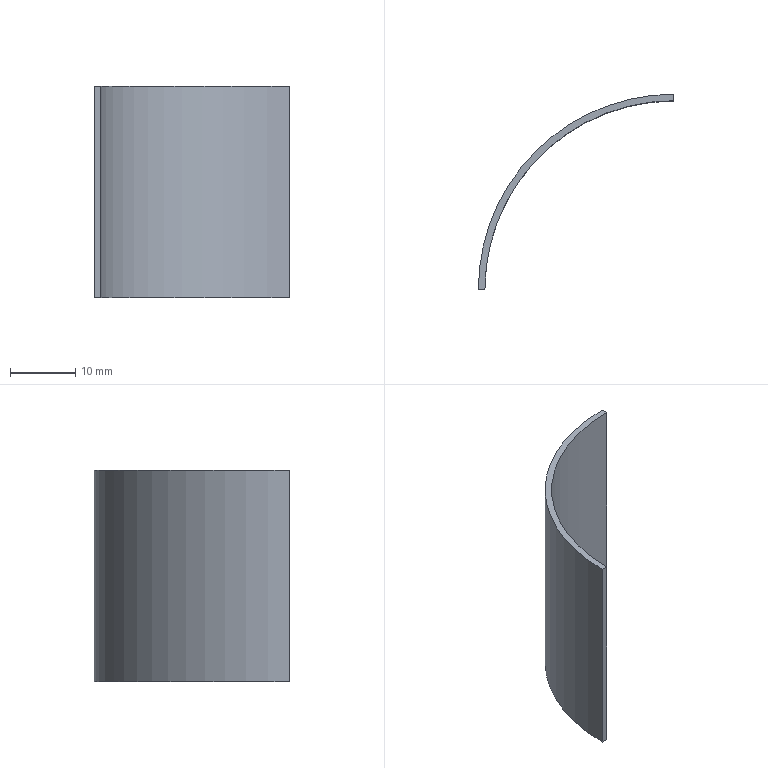Component | SolidWorks | Mirror_w3-2 | 1 solid | 6 faces | box 30 x 30 x 32.5 mm | volume 1506 mm3 | plane 4 | cylinder 2 | commonest cylinder face diameters 60 x1 58 x1
STEP:
#1=COLOUR_RGB('',0.7922,0.8196,0.9333);
#2=FILL_AREA_STYLE_COLOUR('',#1);
#3=FILL_AREA_STYLE('',(#2));
#4=SURFACE_STYLE_FILL_AREA(#3);
#5=SURFACE_SIDE_STYLE('',(#4));
#6=SURFACE_STYLE_USAGE(.BOTH.,#5);
#7=PRESENTATION_STYLE_ASSIGNMENT((#6));
#8=CARTESIAN_POINT('',(-9.843,28.376,-1.28));
#9=VERTEX_POINT('',#8);
#10=CARTESIAN_POINT('',(-8.661,29.557,-1.28));
#11=VERTEX_POINT('',#10);
#12=CARTESIAN_POINT('',(-8.661,28.376,-1.28));
#13=DIRECTION('',(0.,-0.,-1.));
#14=DIRECTION('',(0.,-1.,0.));
#15=AXIS2_PLACEMENT_3D('',#12,#13,#14);
#16=CIRCLE('',#15,1.181);
#17=EDGE_CURVE('',#9,#11,#16,.T.);
#18=ORIENTED_EDGE('',*,*,#17,.F.);
#19=CARTESIAN_POINT('',(-9.843,28.376,-0.));
#20=VERTEX_POINT('',#19);
#21=CARTESIAN_POINT('',(-9.843,28.376,-0.));
#22=DIRECTION('',(0.,-0.,-1.));
#23=VECTOR('',#22,39.37);
#24=LINE('',#21,#23);
#25=EDGE_CURVE('',#20,#9,#24,.T.);
#26=ORIENTED_EDGE('',*,*,#25,.F.);
#27=CARTESIAN_POINT('',(-8.661,29.557,-0.));
#28=VERTEX_POINT('',#27);
#29=CARTESIAN_POINT('',(-8.661,28.376,-0.));
#30=DIRECTION('',(0.,-0.,-1.));
#31=DIRECTION('',(0.,-1.,0.));
#32=AXIS2_PLACEMENT_3D('',#29,#30,#31);
#33=CIRCLE('',#32,1.181);
#34=EDGE_CURVE('',#20,#28,#33,.T.);
#35=ORIENTED_EDGE('',*,*,#34,.T.);
#36=CARTESIAN_POINT('',(-8.661,29.557,-0.));
#37=DIRECTION('',(0.,-0.,-1.));
#38=VECTOR('',#37,39.37);
#39=LINE('',#36,#38);
#40=EDGE_CURVE('',#28,#11,#39,.T.);
#41=ORIENTED_EDGE('',*,*,#40,.T.);
#42=EDGE_LOOP('',(#18,#26,#35,#41));
#43=FACE_OUTER_BOUND('',#42,.T.);
#44=CARTESIAN_POINT('',(-8.661,28.376,-0.));
#45=DIRECTION('',(0.,-0.,-1.));
#46=DIRECTION('',(0.,1.,0.));
#47=AXIS2_PLACEMENT_3D('',#44,#45,#46);
#48=CYLINDRICAL_SURFACE('',#47,1.181);
#49=ADVANCED_FACE('',(#43),#48,.T.);
#50=CARTESIAN_POINT('',(-8.661,29.518,-1.28));
#51=VERTEX_POINT('',#50);
#52=CARTESIAN_POINT('',(-8.661,29.518,-1.28));
#53=DIRECTION('',(0.,1.,-0.));
#54=VECTOR('',#53,39.37);
#55=LINE('',#52,#54);
#56=EDGE_CURVE('',#51,#11,#55,.T.);
#57=ORIENTED_EDGE('',*,*,#56,.T.);
#58=ORIENTED_EDGE('',*,*,#40,.F.);
#59=CARTESIAN_POINT('',(-8.661,29.518,-0.));
#60=VERTEX_POINT('',#59);
#61=CARTESIAN_POINT('',(-8.661,29.518,-0.));
#62=DIRECTION('',(0.,1.,-0.));
#63=VECTOR('',#62,39.37);
#64=LINE('',#61,#63);
#65=EDGE_CURVE('',#60,#28,#64,.T.);
#66=ORIENTED_EDGE('',*,*,#65,.F.);
#67=CARTESIAN_POINT('',(-8.661,29.518,-0.));
#68=DIRECTION('',(0.,-0.,-1.));
#69=VECTOR('',#68,39.37);
#70=LINE('',#67,#69);
#71=EDGE_CURVE('',#60,#51,#70,.T.);
#72=ORIENTED_EDGE('',*,*,#71,.T.);
#73=EDGE_LOOP('',(#57,#58,#66,#72));
#74=FACE_OUTER_BOUND('',#73,.T.);
#75=CARTESIAN_POINT('',(-8.661,29.518,-0.));
#76=DIRECTION('',(1.,-0.,0.));
#77=DIRECTION('',(-0.,-1.,0.));
#78=AXIS2_PLACEMENT_3D('',#75,#76,#77);
#79=PLANE('',#78);
#80=ADVANCED_FACE('',(#74),#79,.T.);
#81=CARTESIAN_POINT('',(-9.803,28.376,-1.28));
#82=VERTEX_POINT('',#81);
#83=CARTESIAN_POINT('',(-8.661,28.376,-1.28));
#84=DIRECTION('',(0.,-0.,-1.));
#85=DIRECTION('',(0.,-1.,0.));
#86=AXIS2_PLACEMENT_3D('',#83,#84,#85);
#87=CIRCLE('',#86,1.142);
#88=EDGE_CURVE('',#82,#51,#87,.T.);
#89=ORIENTED_EDGE('',*,*,#88,.T.);
#90=ORIENTED_EDGE('',*,*,#71,.F.);
#91=CARTESIAN_POINT('',(-9.803,28.376,-0.));
#92=VERTEX_POINT('',#91);
#93=CARTESIAN_POINT('',(-8.661,28.376,-0.));
#94=DIRECTION('',(0.,-0.,-1.));
#95=DIRECTION('',(0.,-1.,0.));
#96=AXIS2_PLACEMENT_3D('',#93,#94,#95);
#97=CIRCLE('',#96,1.142);
#98=EDGE_CURVE('',#92,#60,#97,.T.);
#99=ORIENTED_EDGE('',*,*,#98,.F.);
#100=CARTESIAN_POINT('',(-9.803,28.376,-0.));
#101=DIRECTION('',(0.,-0.,-1.));
#102=VECTOR('',#101,39.37);
#103=LINE('',#100,#102);
#104=EDGE_CURVE('',#92,#82,#103,.T.);
#105=ORIENTED_EDGE('',*,*,#104,.T.);
#106=EDGE_LOOP('',(#89,#90,#99,#105));
#107=FACE_OUTER_BOUND('',#106,.T.);
#108=CARTESIAN_POINT('',(-8.661,28.376,-0.));
#109=DIRECTION('',(0.,-0.,-1.));
#110=DIRECTION('',(0.,1.,0.));
#111=AXIS2_PLACEMENT_3D('',#108,#109,#110);
#112=CYLINDRICAL_SURFACE('',#111,1.142);
#113=ADVANCED_FACE('',(#107),#112,.F.);
#114=CARTESIAN_POINT('',(-9.843,28.376,-1.28));
#115=DIRECTION('',(1.,-0.,0.));
#116=VECTOR('',#115,39.37);
#117=LINE('',#114,#116);
#118=EDGE_CURVE('',#9,#82,#117,.T.);
#119=ORIENTED_EDGE('',*,*,#118,.T.);
#120=ORIENTED_EDGE('',*,*,#104,.F.);
#121=CARTESIAN_POINT('',(-9.843,28.376,-0.));
#122=DIRECTION('',(1.,-0.,0.));
#123=VECTOR('',#122,39.37);
#124=LINE('',#121,#123);
#125=EDGE_CURVE('',#20,#92,#124,.T.);
#126=ORIENTED_EDGE('',*,*,#125,.F.);
#127=ORIENTED_EDGE('',*,*,#25,.T.);
#128=EDGE_LOOP('',(#119,#120,#126,#127));
#129=FACE_OUTER_BOUND('',#128,.T.);
#130=CARTESIAN_POINT('',(-9.843,28.376,-0.));
#131=DIRECTION('',(-0.,-1.,-0.));
#132=DIRECTION('',(-1.,0.,-0.));
#133=AXIS2_PLACEMENT_3D('',#130,#131,#132);
#134=PLANE('',#133);
#135=ADVANCED_FACE('',(#129),#134,.T.);
#136=ORIENTED_EDGE('',*,*,#34,.F.);
#137=ORIENTED_EDGE('',*,*,#125,.T.);
#138=ORIENTED_EDGE('',*,*,#98,.T.);
#139=ORIENTED_EDGE('',*,*,#65,.T.);
#140=EDGE_LOOP('',(#136,#137,#138,#139));
#141=FACE_OUTER_BOUND('',#140,.T.);
#142=CARTESIAN_POINT('',(-8.661,28.376,-0.));
#143=DIRECTION('',(-0.,0.,1.));
#144=DIRECTION('',(-0.,-1.,-0.));
#145=AXIS2_PLACEMENT_3D('',#142,#143,#144);
#146=PLANE('',#145);
#147=ADVANCED_FACE('',(#141),#146,.T.);
#148=ORIENTED_EDGE('',*,*,#17,.T.);
#149=ORIENTED_EDGE('',*,*,#56,.F.);
#150=ORIENTED_EDGE('',*,*,#88,.F.);
#151=ORIENTED_EDGE('',*,*,#118,.F.);
#152=EDGE_LOOP('',(#148,#149,#150,#151));
#153=FACE_OUTER_BOUND('',#152,.T.);
#154=CARTESIAN_POINT('',(-8.661,28.376,-1.28));
#155=DIRECTION('',(-0.,0.,1.));
#156=DIRECTION('',(-0.,-1.,-0.));
#157=AXIS2_PLACEMENT_3D('',#154,#155,#156);
#158=PLANE('',#157);
#159=ADVANCED_FACE('',(#153),#158,.F.);
#160=CLOSED_SHELL('',(#49,#80,#113,#135,#147,#159));
#161=MANIFOLD_SOLID_BREP('',#160);
#162=STYLED_ITEM('',(#7),#161);
#163=(LENGTH_UNIT()NAMED_UNIT(*)SI_UNIT($,.METRE.));
#164=LENGTH_MEASURE_WITH_UNIT(LENGTH_MEASURE(0.0254),#163);
#165=DIMENSIONAL_EXPONENTS(1.,0.,0.,0.,0.,0.,0.);
#166=(CONVERSION_BASED_UNIT('',#164)LENGTH_UNIT()NAMED_UNIT(#165));
#167=UNCERTAINTY_MEASURE_WITH_UNIT(LENGTH_MEASURE(0.00001),#166,'','');
#168=(NAMED_UNIT(*)PLANE_ANGLE_UNIT()SI_UNIT($,.RADIAN.));
#169=(NAMED_UNIT(*)SI_UNIT($,.STERADIAN.)SOLID_ANGLE_UNIT());
#170=(GEOMETRIC_REPRESENTATION_CONTEXT(3)GLOBAL_UNCERTAINTY_ASSIGNED_CONTEXT((#167))GLOBAL_UNIT_ASSIGNED_CONTEXT((#166,#168,#169))REPRESENTATION_CONTEXT('',''));
#171=MECHANICAL_DESIGN_GEOMETRIC_PRESENTATION_REPRESENTATION('',(#162),#170);
#172=CARTESIAN_POINT('',(0.,0.,0.));
#173=DIRECTION('',(0.,0.,1.));
#174=DIRECTION('',(1.,0.,0.));
#175=AXIS2_PLACEMENT_3D('',#172,#173,#174);
#176=(LENGTH_UNIT()NAMED_UNIT(*)SI_UNIT($,.METRE.));
#177=LENGTH_MEASURE_WITH_UNIT(LENGTH_MEASURE(0.0254),#176);
#178=DIMENSIONAL_EXPONENTS(1.,0.,0.,0.,0.,0.,0.);
#179=(CONVERSION_BASED_UNIT('',#177)LENGTH_UNIT()NAMED_UNIT(#178));
#180=UNCERTAINTY_MEASURE_WITH_UNIT(LENGTH_MEASURE(0.00001),#179,'','');
#181=(NAMED_UNIT(*)PLANE_ANGLE_UNIT()SI_UNIT($,.RADIAN.));
#182=(NAMED_UNIT(*)SI_UNIT($,.STERADIAN.)SOLID_ANGLE_UNIT());
#183=(GEOMETRIC_REPRESENTATION_CONTEXT(3)GLOBAL_UNCERTAINTY_ASSIGNED_CONTEXT((#180))GLOBAL_UNIT_ASSIGNED_CONTEXT((#179,#181,#182))REPRESENTATION_CONTEXT('',''));
#184=ADVANCED_BREP_SHAPE_REPRESENTATION('',(#161,#175),#183);
#185=PRESENTATION_LAYER_ASSIGNMENT('','',(#162));